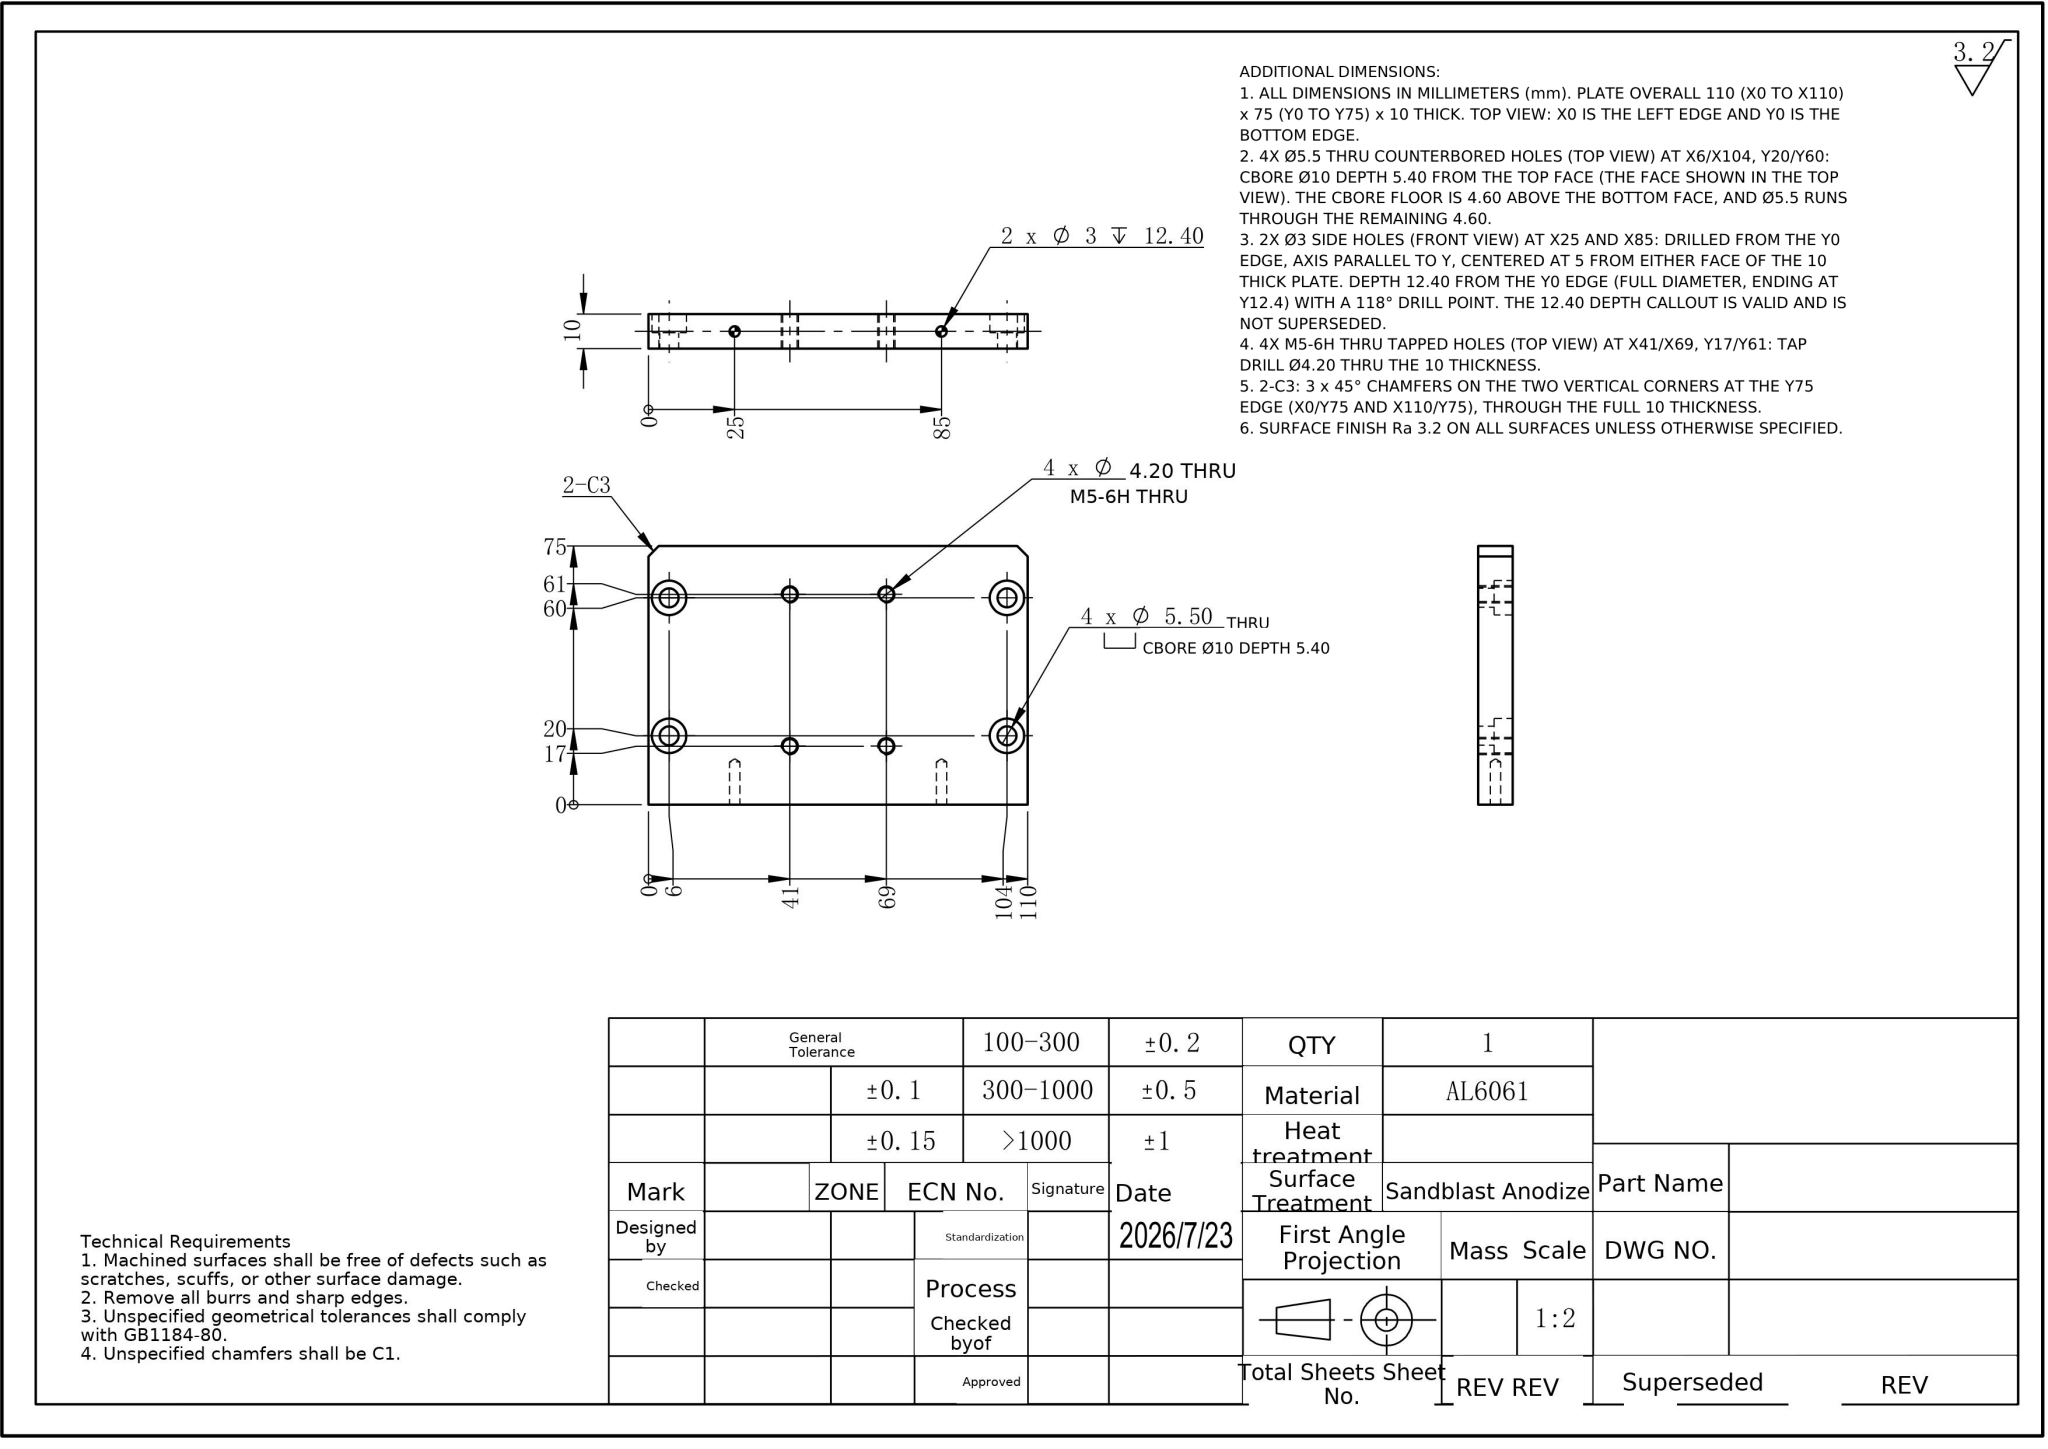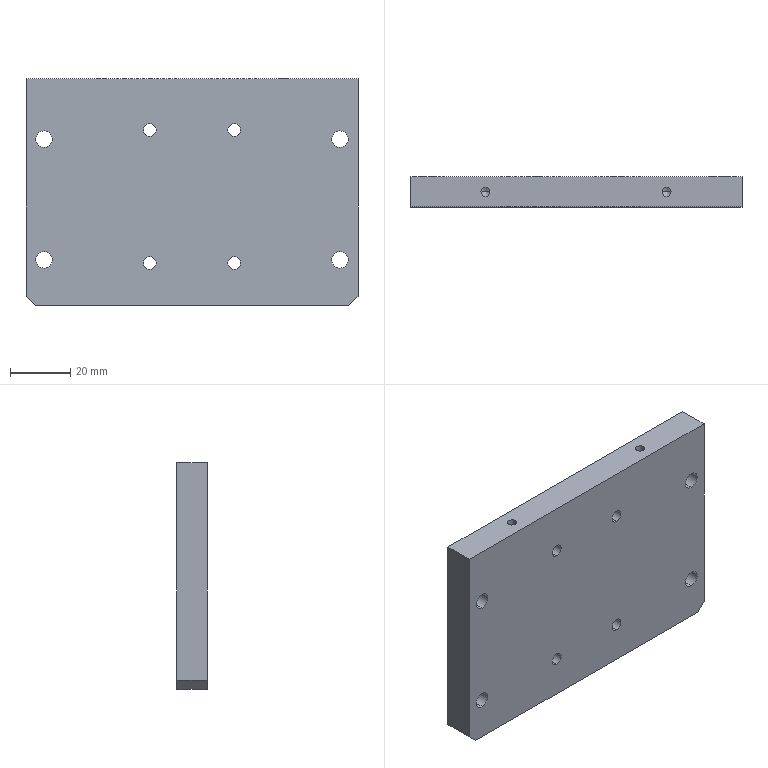Part | NX | mm | 1 solid | 44 faces | box 110 x 10 x 75 mm | volume 79543 mm3 | cylinder 28 | plane 12 | cone 4 | commonest cylinder face diameters 10 x8 5.5 x8 4.2 x8 3 x4